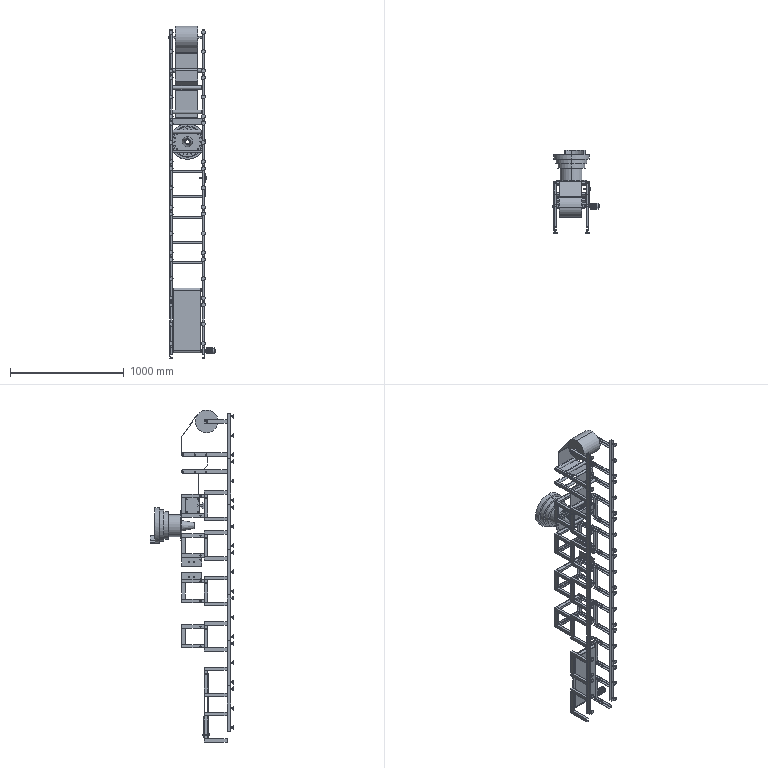Assembly | SolidWorks | mm | 152 component files | 155 solids | 2116 faces | box 413 x 734 x 2923.33 mm | volume 22054020 mm3 | plane 1428 | cylinder 592 | cone 96 | commonest cylinder face diameters 10 x310 35 x84 5 x52 8 x52 30 x33 15 x10 26 x5 34 x5
Bill of materials:
Copy(2)CopyOfPart3 | 4 |  | Straight channel (C/U-section) profile with thin uniform walls, shown standing vertically; constant cross-section along its length with plain square-cut ends.
Copy_of_Copy_of_Part3 | 8 |  | Long, shallow channel (U-section) profile with thin walls; the web is wide and the flanges are short. Constant section, plain ends.
Copy_of_Copy_of_Part4 | 12 |  | Straight channel (C-section) profile, deeper than it is wide, with thin uniform walls and plain square-cut ends; no holes visible.
Copy_of_Part3 | 14 |  | Vertical channel (C-section) profile with thin uniform walls and a single round through-hole in the web near one end.
Copy_of_Part3 | 1 |  | Straight C-section (channel) profile: a flat web with two parallel flanges, cut square at both ends, with one small round through-hole near one end.
Copy_of_Part4 | 1 |  | Straight channel (C-section) profile with thin walls and one round through-hole in the web near one end.
Mirror Copy (2) Copy of Part3^Assembly2 | 4 |  | Straight C-section channel with square-cut ends and no visible holes or cutouts.
Mirror Part3^Assembly2 | 7 |  | Long, slender C-section channel with square-cut ends and three round holes spaced along one face.
Mirror Part4^Assembly2 | 2 |  | Long channel-like or strip-like part with one square-cut open end and one rounded (semicircular) end. A side view shows three small round holes along its length, one of them centered in the rounded end.
Mirror Part8^Assembly2 | 7 |  | Axisymmetric headed pin: a large thin circular disc, a conical (frustum) transition, and a smaller cylindrical shank with a plain flat end.
Mirror Part81^Assembly2 | 7 |  | Axisymmetric headed pin: a large circular disc head, a conical transition, and a cylindrical shank. It looks identical to unnamed part.
Mirror Part82^Assembly2 | 7 |  | Axisymmetric headed pin: a large circular disc head, a conical transition, and a cylindrical shank. It looks identical to parts 4 and 5.
MirrorCopy of Copy of Part4^Assembly2 | 12 |  | Straight C-section channel with square-cut ends and one small round hole in a flange, part way along its length.
MirrorCopy of Part3^Assembly2 | 5 |  | Straight C-section channel with square-cut ends and one small round hole near one end. It looks the same as unnamed part except the hole appears at the opposite end in the view.
MirrorCopy of Part31^Assembly2 | 4 |  | Straight C-section channel with square-cut ends and one round hole in the web near one end.
MirrorCopy of Part33^Assembly2 | 4 |  | Straight C-section channel with one round hole in the web near one end. It looks identical to unnamed part.
MirrorCopy of Part4^Assembly2 | 1 |  | Straight C-section channel with one round hole in the web near the opposite end from parts 9 and 10. The hole looks somewhat larger.
Part1^Assembly2 | 1 |  | Thin, nearly square flat plate with four round through-holes near the corners and one rectangular notch cut into one edge.
Part10 | 1 |  | Cylindrical body with many shallow longitudinal grooves/ribs around its outer surface. One end has a stepped shaft (two smaller diameters). The other end has a shorter stepped boss ending in a conical taper. The end view shows small radial projections spaced around the rim.
Part2^Assembly2 | 1 |  | Two separate, thin, rectangular flat plates in one part, set side by side and parallel. Each has three round through-holes: two near the middle in line and one near a corner. The two hole layouts mirror each other.
Part20 | 1 |  | Long rectangular bar with round holes near each end on one long face. One end has a stepped/notched profile. The end view shows a cross-section with tapered (chamfered or trapezoidal) sides and a small stepped protrusion. One side view shows a raised thin strip and small cylindrical features, plus regularly spaced light marks along the length.
Part21 | 2 |  | Solid cylindrical pin with chamfered ends and a flat, wedge-shaped tab or fin sticking out sideways along the middle part of its length.
Part22 | 2 |  | Long, slender, straight bar with a square or near-square solid cross-section and plain ends.
Part23 | 1 |  | Stepped cylindrical shaft: a short larger-diameter section at one end, a long smaller-diameter middle section, and a flat rectangular tab at the other end with a round cross-hole.
Part24 | 1 |  | Mostly revolved stepped body. From one end to the other it has a hollow conical nozzle, a thin flange drilled with a circle of small holes, a cylindrical barrel, and then three cylindrical steps that get larger toward the far end. A small block sticks out sideways, off-axis, at the large end.
Part3^Assembly2 | 1 |  | Headed pin: a plain cylindrical shank with a larger coaxial disc-shaped head at one end.
Part3 | 7 |  | Long straight channel with a C/U-shaped cross-section, square-cut at both ends, with three round holes evenly spaced along one wall.
Part4 | 2 |  | Long straight channel with a C-shaped cross-section. One end is rounded (semicircular in side profile) and the other is square-cut. The web has three round holes, mostly toward the rounded end.
Part5 | 9 |  | Stepped cylindrical shaft: a long, larger-diameter body with a smaller-diameter coaxial journal at each end, symmetric end to end.
Part6 | 1 |  | Formed thin strip with several bends and a joggled lower leg, shown with a solid cylinder whose thin coaxial pin sticks out from both ends. The strip starts at a tangent near the cylinder.
Part7 | 1 |  | Straight thin-walled flat-oval (obround) hollow tube with open ends.
Part8 | 21 |  | Revolved headed pin: a wide, thin disc head, a conical frustum taper, then a smaller cylindrical shank.
Mates:
1. coincident | Part3-1 face at (152, 30, 398.45) dir (0, 1, 0) | Part4-1 face at (152, 30, -274.216) dir (0, -1, 0)
2. coincident | Part3-1 face at (152, 0, 398.45) dir (1, 0, 0) | Part4-1 face at (152, 430, -100.396) dir (1, 0, 0)
3. distance | Part3-1 face at (150, 0, 398.45) dir (-1, 0, 0) | assembly plane at (0, 0, 0) dir (1, 0, 0)
4. coincident | Part3-1 face at (152, 0, 398.45) dir (0, -1, 0) | assembly plane at (0, 0, 0) dir (0, 1, 0)
5. concentric | Part4-1 face at (98, 415, -115.396) dir (1, 0, 0) r 15 | Part5-1 face at (152, 415, -115.396) dir (-1, 0, 0) r 5
6. coincident | Part4-1 face at (152, 430, -100.396) dir (1, 0, 0) | Part5-1 face at (152, 415, -115.396) dir (1, 0, 0)
7. concentric | Part4-4 face at (98, 415, 34.604) dir (1, 0, 0) r 15 | Part5-2 face at (152, 415, 34.604) dir (-1, 0, 0) r 5
8. coincident | Part4-4 face at (152, 430, 49.604) dir (1, 0, 0) | Part5-2 face at (152, 415, 34.604) dir (1, 0, 0)
9. coincident | Part3-1 face at (152, 0, 398.45) dir (1, 0, 0) | Copy_of_Part4-1 face at (152, 230, 341.534) dir (1, 0, 0)
10. coincident | Part3-1 face at (152, 30, 398.45) dir (0, 1, 0) | Copy_of_Part4-1 face at (152, 30, 167.715) dir (0, -1, 0)
11. concentric | Copy_of_Part4-1 face at (-102, 209.97, 327.241) dir (1, 0, 0) r 7.5 | Part6-1 face at (-164, 209.97, 327.241) dir (1, 0, 0) r 7.5
12. coincident | Copy_of_Part4-1 face at (152, 230, 341.534) dir (1, 0, 0) | Part6-1 face at (152, 209.97, 327.241) dir (1, 0, 0)
13. concentric | Part5-3 face at (152, 315, -115.396) dir (-1, 0, 0) r 5 | Mirror Part4^Assembly2-2 edge at (-150, 315, -115.396) dir (1, 0, 0) r 5
14. coincident | Mirror Part4^Assembly2-2 face at (-152, 430, -100.396) dir (-1, 0, 0) | Part5-3 face at (-152, 315, -115.396) dir (-1, 0, 0)
15. concentric | Part5-4 edge at (-152, 215, -115.396) dir (1, 0, 0) r 5 | Mirror Part4^Assembly2-2 face at (-98, 215, -115.396) dir (-1, 0, 0) r 5
16. coincident | Mirror Part4^Assembly2-2 face at (-152, 430, -100.396) dir (-1, 0, 0) | Part5-4 face at (-152, 215, -115.396) dir (-1, 0, 0)
17. concentric | Part3-1 face at (142, 5, 371.683) dir (0, -1, 0) r 5 | Part8-1 face at (142, 2, 371.683) dir (0, -1, 0) r 5
18. coincident | Part3-1 face at (152, 2, 398.45) dir (0, 1, 0) | Part8-1 face at (142, 2, 371.683) dir (0, 1, 0)
19. coincident | Part3-3 face at (152, 0, -1.55) dir (1, 0, 0) | Copy_of_Copy_of_Part4-1 face at (152, 230, -286.092) dir (1, 0, 0)
20. coincident | Part3-3 face at (152, 30, -1.55) dir (0, 1, 0) | Copy_of_Copy_of_Part4-1 face at (152, 30, -459.911) dir (0, -1, 0)
21. coincident | Copy_of_Copy_of_Part4-1 face at (152, 230, -286.092) dir (1, 0, 0) | Copy_of_Part3-1 face at (152, 200, -316.092) dir (1, 0, 0)
22. coincident | Copy_of_Copy_of_Part4-1 face at (132, 230, -316.092) dir (0, 0, -1) | Copy_of_Part3-1 face at (152, 214.124, -316.092) dir (0, 0, 1)
23. coincident | Copy_of_Copy_of_Part4-1 face at (152, 230, -459.911) dir (0, 1, 0) | Copy_of_Part3-1 face at (152, 230, -316.092) dir (0, 1, 0)
24. coincident | Copy_of_Copy_of_Part4-1 face at (132, 230, -314.092) dir (0, 0, 1) | Copy_of_Part3-14 face at (152, 230, -314.092) dir (0, 0, 1)
25. coincident | Copy_of_Copy_of_Part4-1 face at (152, 230, -286.092) dir (1, 0, 0) | Copy_of_Part3-14 face at (152, 230, -344.092) dir (1, 0, 0)
26. coincident | Copy_of_Part3-1 face at (152, 230, -316.092) dir (0, 1, 0) | Copy_of_Part3-14 face at (152, 230, -329.968) dir (0, -1, 0)
27. coincident | Copy_of_Part3-14 face at (152, 230, -316.092) dir (0, 0, -1) | Copy_of_Copy_of_Part3-1 face at (-150, 400, -316.092) dir (0, 0, 1)
28. coincident | Copy_of_Part3-14 face at (150, 230, -344.092) dir (-1, 0, 0) | Copy_of_Copy_of_Part3-1 face at (150, 414.124, -316.092) dir (1, 0, 0)
29. coincident | Copy_of_Part3-14 face at (152, 430, -329.968) dir (0, 1, 0) | Copy_of_Copy_of_Part3-1 face at (-150, 430, -316.092) dir (0, 1, 0)
30. coincident | Copy_of_Part3-14 face at (152, 230, -344.092) dir (1, 0, 0) | Copy(2)CopyOfPart3-1 face at (152, 400, -344.092) dir (1, 0, 0)
31. coincident | Copy_of_Copy_of_Part3-1 face at (-150, 430, -316.092) dir (0, 1, 0) | Copy(2)CopyOfPart3-1 face at (152, 430, -344.092) dir (0, 1, 0)
32. coincident | Copy_of_Part3-14 face at (152, 230, -344.092) dir (0, 0, -1) | Copy(2)CopyOfPart3-1 face at (152, 414.124, -344.092) dir (0, 0, 1)
33. coincident | Copy_of_Part3-1 face at (152, 200, -316.092) dir (1, 0, 0) | Copy_of_Part3-24 face at (152, 230, -518.092) dir (1, 0, 0)
34. coincident | Copy_of_Copy_of_Part4-3 face at (132, 230, -518.092) dir (0, 0, -1) | Copy_of_Part3-24 face at (152, 230, -518.092) dir (0, 0, -1)
35. coincident | Copy_of_Part3-1 face at (152, 230, -316.092) dir (0, 1, 0) | Copy_of_Part3-24 face at (152, 230, -503.968) dir (0, -1, 0)
36. coincident | Copy_of_Part3-24 face at (150, 230, -518.092) dir (-1, 0, 0) | Copy_of_Copy_of_Part3-11 face at (150, 414.124, -516.092) dir (1, 0, 0)
37. coincident | Copy_of_Part3-24 face at (152, 230, -516.092) dir (0, 0, 1) | Copy_of_Copy_of_Part3-11 face at (150, 400, -516.092) dir (0, 0, -1)
38. coincident | Copy(2)CopyOfPart3-1 face at (152, 430, -344.092) dir (0, 1, 0) | Copy_of_Copy_of_Part3-11 face at (150, 430, -516.092) dir (0, 1, 0)
39. concentric | Copy_of_Part3-14 edge at (152, 263.719, -329.968) dir (1, 0, 0) r 5 | Part5-5 face at (152, 263.719, -329.968) dir (-1, 0, 0) r 5
40. coincident | Copy_of_Part3-14 face at (152, 230, -344.092) dir (1, 0, 0) | Part5-5 face at (152, 263.719, -329.968) dir (1, 0, 0)
41. concentric | Copy_of_Part3-24 edge at (152, 263.719, -503.968) dir (1, 0, 0) r 5 | Part5-6 face at (152, 263.719, -503.968) dir (-1, 0, 0) r 5
42. coincident | Copy_of_Part3-24 face at (152, 230, -518.092) dir (1, 0, 0) | Part5-6 face at (152, 263.719, -503.968) dir (1, 0, 0)
43. width | Copy_of_Part3-1 face at (152, 200, -316.092) dir (1, 0, 0) | MirrorCopy of Part3^Assembly2-2 face at (-152, 200, -316.092) dir (-1, 0, 0) | Part20-1 face at (-145.5, 156.346, 23.268) dir (-1, 0, 0) | Part20-1 face at (145.5, 156.346, 23.268) dir (1, 0, 0)
44. concentric | Part21-1 face at (153.525, 273, -412.433) dir (0, -1, 0) r 4 | Part22-1 face at (153.525, 280.245, -412.433) dir (0, -1, 0) r 2.5
45. parallel | Part20-1 face at (145.5, 156.346, 23.268) dir (1, 0, 0) | Part22-1 face at (154.105, 285.245, -414.865) dir (1, 0, 0)
46. coincident | Part20-1 face at (145.5, 156.346, 23.268) dir (1, 0, 0) | Part21-1 face at (145.5, 243, -419.26) dir (-1, 0, 0)
47. coincident | Copy_of_Part3-1 face at (152, 230, -316.092) dir (0, 1, 0) | Part21-1 face at (153.525, 230, -412.433) dir (0, -1, 0)
48. coincident | Part22-1 face at (152.794, 285.245, -414.865) dir (-1, 0, 0) | Part23-1 face at (152.794, -25.683, -135.592) dir (1, 0, 0)
49. coincident | Part22-1 face at (154.105, 285.245, -410.043) dir (0, 0, 1) | Part23-1 face at (-152.786, 285.245, -410.043) dir (0, 0, 1)
50. coincident | Part22-1 face at (-113.999, 285.245, -572.459) dir (0, 1, 0) | Part23-1 face at (-152.786, 285.245, -410.043) dir (0, 1, 0)
51. coincident | Part20-1 edge at (145.5, 246.054, -405.633) dir (0, 1, 0) | Part21-1 edge at (145.5, 243, -405.633) dir (0, 1, 0)
52. width | Copy_of_Part3-24 face at (152, 230, -518.092) dir (0, 0, -1) | Copy_of_Part3-14 face at (152, 230, -314.092) dir (0, 0, 1) | Part20-1 face at (-145.5, 230, -388.598) dir (0, 0, 1) | Part20-1 face at (-145.5, 246.054, -443.586) dir (0, 0, -1)
53. distance | Copy_of_Copy_of_Part4-1 face at (132, 230, -286.092) dir (0, 0, 1) | Part4-1 face at (132, 430, -130.396) dir (0, 0, -1)
54. coincident | Copy_of_Copy_of_Part3-12 face at (150, 430, -866.092) dir (0, 1, 0) | Part24-1 face at (2.194, 430, -591.092) dir (0, -1, 0)
55. concentric | Copy_of_Part3-12 edge at (152, 214.124, -1899.811) dir (1, 0, 0) r 5 | Part5-7 face at (152, 214.124, -1899.811) dir (-1, 0, 0) r 5
56. coincident | Copy_of_Copy_of_Part4-20 face at (152, 230, -1836.092) dir (1, 0, 0) | Part5-7 face at (152, 214.124, -1899.811) dir (1, 0, 0)
57. concentric | Copy_of_Part3-13 edge at (152, 214.124, -2156.717) dir (1, 0, 0) r 5 | assembly face at (152, 214.124, -2156.717) dir (-1, 0, 0) r 5
58. coincident | Copy_of_Copy_of_Part4-15 face at (152, 230, -2639.911) dir (0, 1, 0) | Copy_of_Part3-28 face at (152, 230, -2466.092) dir (0, 1, 0)
59. coincident | Copy_of_Copy_of_Part4-15 face at (152, 230, -2466.092) dir (1, 0, 0) | Copy_of_Part3-28 face at (152, 230, -2466.092) dir (1, 0, 0)
60. coincident | Copy_of_Copy_of_Part4-15 face at (132, 230, -2466.092) dir (0, 0, 1) | Copy_of_Part3-28 face at (152, 215.876, -2466.092) dir (0, 0, -1)
61. coincident | MirrorCopy of Copy of Part4^Assembly2-16 face at (-152, 230, -2639.911) dir (0, 1, 0) | Copy_of_Part3-29 face at (-152, 230, -2466.092) dir (0, 1, 0)
62. coincident | MirrorCopy of Copy of Part4^Assembly2-16 face at (-132, 230, -2466.092) dir (0, 0, 1) | Copy_of_Part3-29 face at (-152, 214.124, -2466.092) dir (0, 0, -1)
63. coincident | MirrorCopy of Copy of Part4^Assembly2-16 face at (-152, 230, -2466.092) dir (-1, 0, 0) | Copy_of_Part3-29 face at (-152, 200, -2466.092) dir (-1, 0, 0)
64. concentric | Copy_of_Part3-28 edge at (152, 215.876, -2432.373) dir (1, 0, 0) r 5 | Part5-9 face at (152, 215.876, -2432.373) dir (-1, 0, 0) r 5
65. coincident | Copy_of_Part3-28 face at (152, 230, -2466.092) dir (1, 0, 0) | Part5-9 face at (152, 215.876, -2432.373) dir (1, 0, 0)
66. concentric | Part4-4 edge at (152, 315, 34.604) dir (1, 0, 0) r 5 | Part5-10 face at (152, 315, 34.604) dir (-1, 0, 0) r 5
67. coincident | Part4-4 face at (152, 430, 49.604) dir (1, 0, 0) | Part5-10 face at (152, 315, 34.604) dir (1, 0, 0)
68. coincident | Copy_of_Part3-14 face at (152, 230, -344.092) dir (1, 0, 0) | Part1^Assembly2-1 face at (152, 65.658, -219.167) dir (1, 0, 0)
69. coincident | Copy_of_Part3-14 face at (152, 230, -344.092) dir (0, 0, -1) | Part1^Assembly2-1 face at (152, 400, -344.092) dir (0, 0, 1)
70. coincident | Copy(2)CopyOfPart3-1 face at (152, 400, -344.092) dir (0, -1, 0) | Part1^Assembly2-1 face at (152, 400, -488.092) dir (0, 1, 0)
71. concentric | Part5-2 face at (127, 415, 34.604) dir (-1, 0, 0) r 15 | Part6-1 face at (-106, 415, 34.604) dir (1, 0, 0) r 17